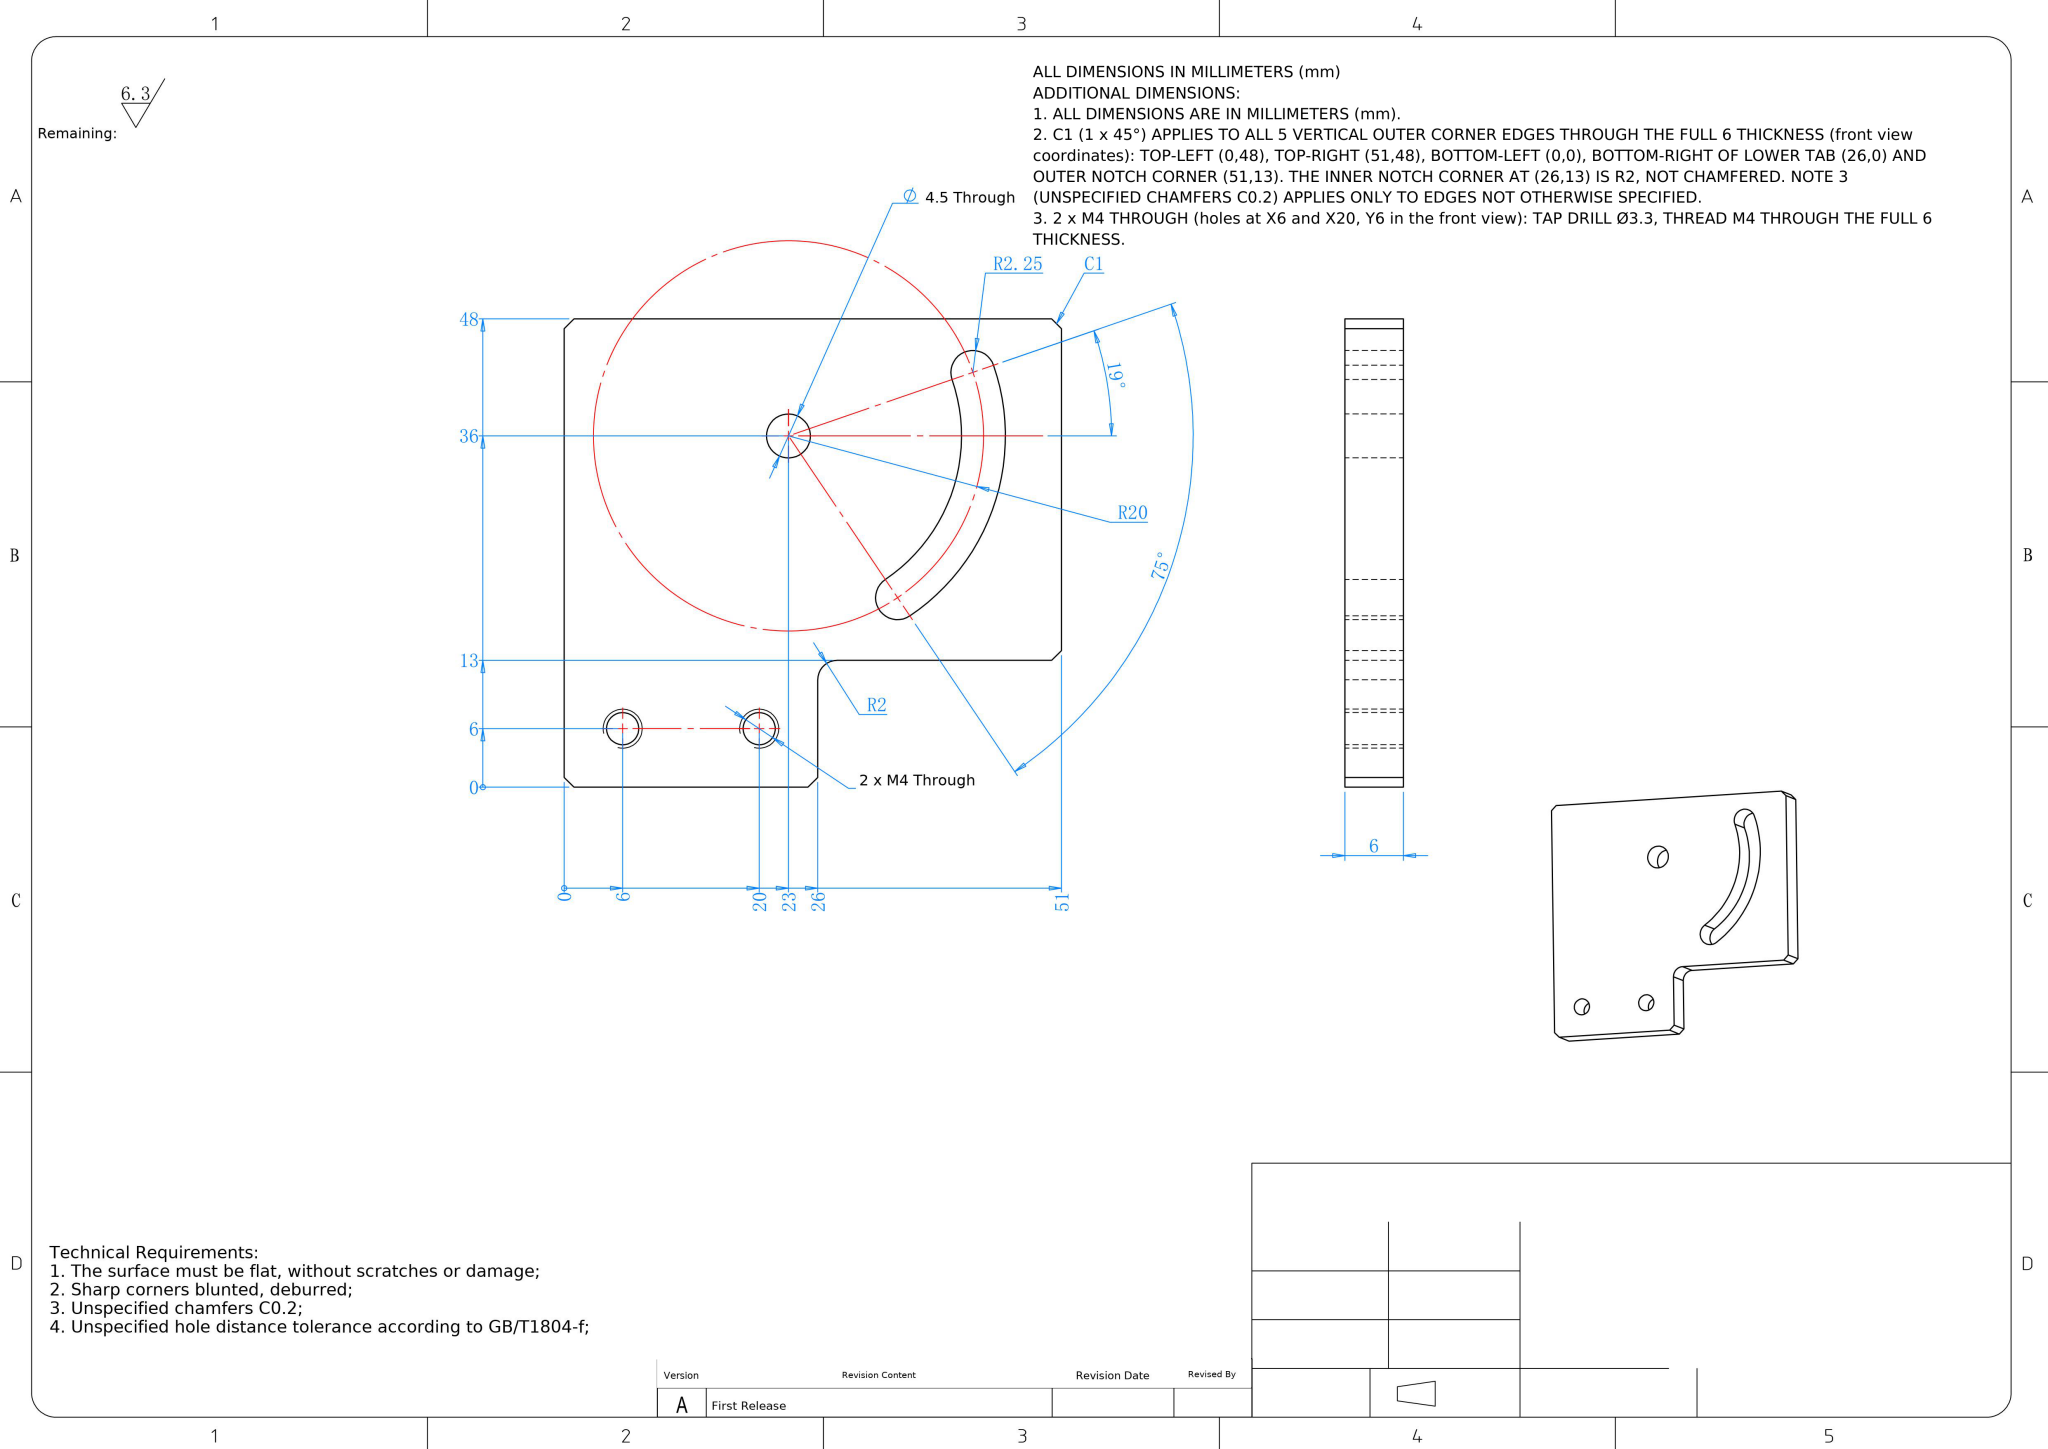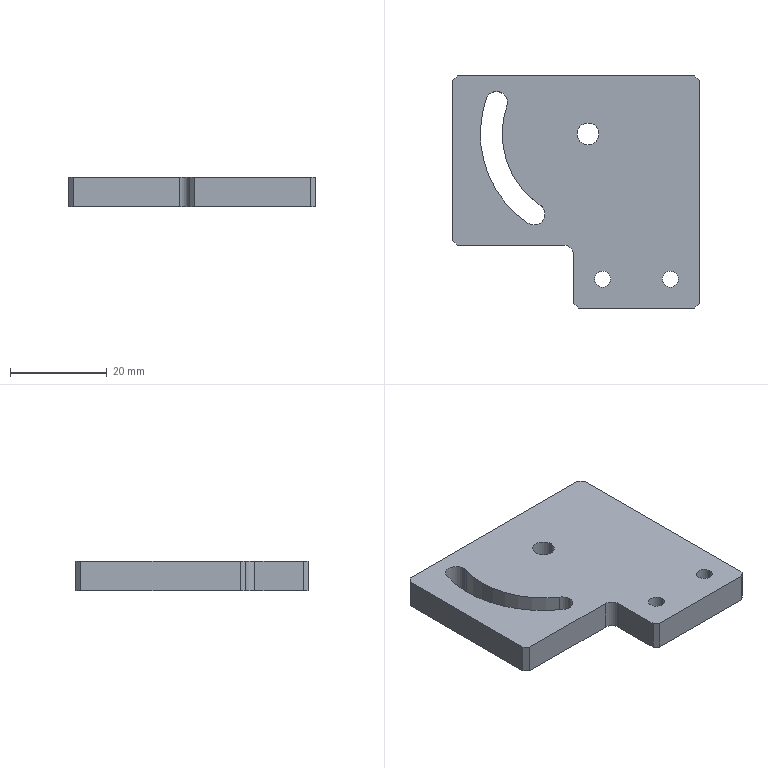Part | NX | mm | Right-Angle Hooked Shelf Bracket 48mm | 1 solid | 26 faces | box 51 x 48 x 6 mm | volume 11728 mm3 | cylinder 13 | plane 13 | commonest cylinder face diameters 4.5 x6 3.3 x4 35.5 x1 44.5 x1 4 x1
STEP:
#1=COLOUR_RGB('',0.7922,0.8196,0.9333);
#2=FILL_AREA_STYLE_COLOUR('',#1);
#3=FILL_AREA_STYLE('',(#2));
#4=SURFACE_STYLE_FILL_AREA(#3);
#5=SURFACE_SIDE_STYLE('',(#4));
#6=SURFACE_STYLE_USAGE(.BOTH.,#5);
#7=PRESENTATION_STYLE_ASSIGNMENT((#6));
#8=CARTESIAN_POINT('',(1.35,-30.,0.));
#9=VERTEX_POINT('',#8);
#10=CARTESIAN_POINT('',(4.65,-30.,0.));
#11=VERTEX_POINT('',#10);
#12=CARTESIAN_POINT('',(3.,-30.,0.));
#13=DIRECTION('',(0.,0.,1.));
#14=DIRECTION('',(1.,0.,0.));
#15=AXIS2_PLACEMENT_3D('',#12,#13,#14);
#16=CIRCLE('',#15,1.65);
#17=EDGE_CURVE('',#9,#11,#16,.T.);
#18=ORIENTED_EDGE('',*,*,#17,.F.);
#19=CARTESIAN_POINT('',(1.35,-30.,6.));
#20=VERTEX_POINT('',#19);
#21=CARTESIAN_POINT('',(1.35,-30.,6.));
#22=DIRECTION('',(0.,0.,1.));
#23=VECTOR('',#22,1000.);
#24=LINE('',#21,#23);
#25=EDGE_CURVE('',#9,#20,#24,.T.);
#26=ORIENTED_EDGE('',*,*,#25,.T.);
#27=CARTESIAN_POINT('',(4.65,-30.,6.));
#28=VERTEX_POINT('',#27);
#29=CARTESIAN_POINT('',(3.,-30.,6.));
#30=DIRECTION('',(0.,0.,1.));
#31=DIRECTION('',(1.,0.,0.));
#32=AXIS2_PLACEMENT_3D('',#29,#30,#31);
#33=CIRCLE('',#32,1.65);
#34=EDGE_CURVE('',#20,#28,#33,.T.);
#35=ORIENTED_EDGE('',*,*,#34,.T.);
#36=CARTESIAN_POINT('',(4.65,-30.,6.));
#37=DIRECTION('',(0.,0.,1.));
#38=VECTOR('',#37,1000.);
#39=LINE('',#36,#38);
#40=EDGE_CURVE('',#11,#28,#39,.T.);
#41=ORIENTED_EDGE('',*,*,#40,.F.);
#42=EDGE_LOOP('',(#18,#26,#35,#41));
#43=FACE_OUTER_BOUND('',#42,.T.);
#44=CARTESIAN_POINT('',(3.,-30.,6.));
#45=DIRECTION('',(0.,0.,1.));
#46=DIRECTION('',(1.,0.,0.));
#47=AXIS2_PLACEMENT_3D('',#44,#45,#46);
#48=CYLINDRICAL_SURFACE('',#47,1.65);
#49=ADVANCED_FACE('',(#43),#48,.F.);
#50=CARTESIAN_POINT('',(15.35,-30.,0.));
#51=VERTEX_POINT('',#50);
#52=CARTESIAN_POINT('',(18.65,-30.,0.));
#53=VERTEX_POINT('',#52);
#54=CARTESIAN_POINT('',(17.,-30.,0.));
#55=DIRECTION('',(0.,0.,1.));
#56=DIRECTION('',(1.,0.,0.));
#57=AXIS2_PLACEMENT_3D('',#54,#55,#56);
#58=CIRCLE('',#57,1.65);
#59=EDGE_CURVE('',#51,#53,#58,.T.);
#60=ORIENTED_EDGE('',*,*,#59,.F.);
#61=CARTESIAN_POINT('',(15.35,-30.,6.));
#62=VERTEX_POINT('',#61);
#63=CARTESIAN_POINT('',(15.35,-30.,6.));
#64=DIRECTION('',(0.,0.,1.));
#65=VECTOR('',#64,1000.);
#66=LINE('',#63,#65);
#67=EDGE_CURVE('',#51,#62,#66,.T.);
#68=ORIENTED_EDGE('',*,*,#67,.T.);
#69=CARTESIAN_POINT('',(18.65,-30.,6.));
#70=VERTEX_POINT('',#69);
#71=CARTESIAN_POINT('',(17.,-30.,6.));
#72=DIRECTION('',(0.,0.,1.));
#73=DIRECTION('',(1.,0.,0.));
#74=AXIS2_PLACEMENT_3D('',#71,#72,#73);
#75=CIRCLE('',#74,1.65);
#76=EDGE_CURVE('',#62,#70,#75,.T.);
#77=ORIENTED_EDGE('',*,*,#76,.T.);
#78=CARTESIAN_POINT('',(18.65,-30.,6.));
#79=DIRECTION('',(0.,0.,1.));
#80=VECTOR('',#79,1000.);
#81=LINE('',#78,#80);
#82=EDGE_CURVE('',#53,#70,#81,.T.);
#83=ORIENTED_EDGE('',*,*,#82,.F.);
#84=EDGE_LOOP('',(#60,#68,#77,#83));
#85=FACE_OUTER_BOUND('',#84,.T.);
#86=CARTESIAN_POINT('',(17.,-30.,6.));
#87=DIRECTION('',(0.,0.,1.));
#88=DIRECTION('',(1.,0.,0.));
#89=AXIS2_PLACEMENT_3D('',#86,#87,#88);
#90=CYLINDRICAL_SURFACE('',#89,1.65);
#91=ADVANCED_FACE('',(#85),#90,.F.);
#92=CARTESIAN_POINT('',(-8.934,-16.581,0.));
#93=VERTEX_POINT('',#92);
#94=CARTESIAN_POINT('',(-9.926,-14.715,0.));
#95=VERTEX_POINT('',#94);
#96=CARTESIAN_POINT('',(-11.184,-16.581,0.));
#97=DIRECTION('',(0.,0.,1.));
#98=DIRECTION('',(-1.,0.,0.));
#99=AXIS2_PLACEMENT_3D('',#96,#97,#98);
#100=CIRCLE('',#99,2.25);
#101=EDGE_CURVE('',#93,#95,#100,.T.);
#102=ORIENTED_EDGE('',*,*,#101,.F.);
#103=CARTESIAN_POINT('',(-8.934,-16.581,6.));
#104=VERTEX_POINT('',#103);
#105=CARTESIAN_POINT('',(-8.934,-16.581,0.));
#106=DIRECTION('',(0.,0.,1.));
#107=VECTOR('',#106,1000.);
#108=LINE('',#105,#107);
#109=EDGE_CURVE('',#93,#104,#108,.T.);
#110=ORIENTED_EDGE('',*,*,#109,.T.);
#111=CARTESIAN_POINT('',(-9.926,-14.715,6.));
#112=VERTEX_POINT('',#111);
#113=CARTESIAN_POINT('',(-11.184,-16.581,6.));
#114=DIRECTION('',(0.,0.,1.));
#115=DIRECTION('',(-1.,0.,0.));
#116=AXIS2_PLACEMENT_3D('',#113,#114,#115);
#117=CIRCLE('',#116,2.25);
#118=EDGE_CURVE('',#104,#112,#117,.T.);
#119=ORIENTED_EDGE('',*,*,#118,.T.);
#120=CARTESIAN_POINT('',(-9.926,-14.715,0.));
#121=DIRECTION('',(0.,0.,1.));
#122=VECTOR('',#121,1000.);
#123=LINE('',#120,#122);
#124=EDGE_CURVE('',#95,#112,#123,.T.);
#125=ORIENTED_EDGE('',*,*,#124,.F.);
#126=EDGE_LOOP('',(#102,#110,#119,#125));
#127=FACE_OUTER_BOUND('',#126,.T.);
#128=CARTESIAN_POINT('',(-11.184,-16.581,0.));
#129=DIRECTION('',(0.,0.,1.));
#130=DIRECTION('',(1.,0.,0.));
#131=AXIS2_PLACEMENT_3D('',#128,#129,#130);
#132=CYLINDRICAL_SURFACE('',#131,2.25);
#133=ADVANCED_FACE('',(#127),#132,.F.);
#134=CARTESIAN_POINT('',(-16.66,6.511,0.));
#135=VERTEX_POINT('',#134);
#136=CARTESIAN_POINT('',(-21.038,7.244,0.));
#137=VERTEX_POINT('',#136);
#138=CARTESIAN_POINT('',(-18.91,6.511,0.));
#139=DIRECTION('',(0.,0.,1.));
#140=DIRECTION('',(1.,0.,0.));
#141=AXIS2_PLACEMENT_3D('',#138,#139,#140);
#142=CIRCLE('',#141,2.25);
#143=EDGE_CURVE('',#135,#137,#142,.T.);
#144=ORIENTED_EDGE('',*,*,#143,.F.);
#145=CARTESIAN_POINT('',(-16.66,6.511,6.));
#146=VERTEX_POINT('',#145);
#147=CARTESIAN_POINT('',(-16.66,6.511,0.));
#148=DIRECTION('',(0.,0.,1.));
#149=VECTOR('',#148,1000.);
#150=LINE('',#147,#149);
#151=EDGE_CURVE('',#135,#146,#150,.T.);
#152=ORIENTED_EDGE('',*,*,#151,.T.);
#153=CARTESIAN_POINT('',(-21.038,7.244,6.));
#154=VERTEX_POINT('',#153);
#155=CARTESIAN_POINT('',(-18.91,6.511,6.));
#156=DIRECTION('',(0.,0.,1.));
#157=DIRECTION('',(1.,0.,0.));
#158=AXIS2_PLACEMENT_3D('',#155,#156,#157);
#159=CIRCLE('',#158,2.25);
#160=EDGE_CURVE('',#146,#154,#159,.T.);
#161=ORIENTED_EDGE('',*,*,#160,.T.);
#162=CARTESIAN_POINT('',(-21.038,7.244,0.));
#163=DIRECTION('',(0.,0.,1.));
#164=VECTOR('',#163,1000.);
#165=LINE('',#162,#164);
#166=EDGE_CURVE('',#137,#154,#165,.T.);
#167=ORIENTED_EDGE('',*,*,#166,.F.);
#168=EDGE_LOOP('',(#144,#152,#161,#167));
#169=FACE_OUTER_BOUND('',#168,.T.);
#170=CARTESIAN_POINT('',(-18.91,6.511,0.));
#171=DIRECTION('',(0.,0.,1.));
#172=DIRECTION('',(1.,0.,0.));
#173=AXIS2_PLACEMENT_3D('',#170,#171,#172);
#174=CYLINDRICAL_SURFACE('',#173,2.25);
#175=ADVANCED_FACE('',(#169),#174,.F.);
#176=CARTESIAN_POINT('',(-2.25,0.,0.));
#177=VERTEX_POINT('',#176);
#178=CARTESIAN_POINT('',(2.25,0.,0.));
#179=VERTEX_POINT('',#178);
#180=CARTESIAN_POINT('',(0.,0.,0.));
#181=DIRECTION('',(0.,0.,1.));
#182=DIRECTION('',(1.,0.,0.));
#183=AXIS2_PLACEMENT_3D('',#180,#181,#182);
#184=CIRCLE('',#183,2.25);
#185=EDGE_CURVE('',#177,#179,#184,.T.);
#186=ORIENTED_EDGE('',*,*,#185,.F.);
#187=CARTESIAN_POINT('',(-2.25,0.,6.));
#188=VERTEX_POINT('',#187);
#189=CARTESIAN_POINT('',(-2.25,0.,6.));
#190=DIRECTION('',(0.,0.,1.));
#191=VECTOR('',#190,1000.);
#192=LINE('',#189,#191);
#193=EDGE_CURVE('',#177,#188,#192,.T.);
#194=ORIENTED_EDGE('',*,*,#193,.T.);
#195=CARTESIAN_POINT('',(2.25,0.,6.));
#196=VERTEX_POINT('',#195);
#197=CARTESIAN_POINT('',(0.,0.,6.));
#198=DIRECTION('',(0.,0.,1.));
#199=DIRECTION('',(1.,0.,0.));
#200=AXIS2_PLACEMENT_3D('',#197,#198,#199);
#201=CIRCLE('',#200,2.25);
#202=EDGE_CURVE('',#188,#196,#201,.T.);
#203=ORIENTED_EDGE('',*,*,#202,.T.);
#204=CARTESIAN_POINT('',(2.25,0.,6.));
#205=DIRECTION('',(0.,0.,1.));
#206=VECTOR('',#205,1000.);
#207=LINE('',#204,#206);
#208=EDGE_CURVE('',#179,#196,#207,.T.);
#209=ORIENTED_EDGE('',*,*,#208,.F.);
#210=EDGE_LOOP('',(#186,#194,#203,#209));
#211=FACE_OUTER_BOUND('',#210,.T.);
#212=CARTESIAN_POINT('',(0.,0.,6.));
#213=DIRECTION('',(0.,0.,1.));
#214=DIRECTION('',(1.,0.,0.));
#215=AXIS2_PLACEMENT_3D('',#212,#213,#214);
#216=CYLINDRICAL_SURFACE('',#215,2.25);
#217=ADVANCED_FACE('',(#211),#216,.F.);
#218=CARTESIAN_POINT('',(-28.,11.,6.));
#219=VERTEX_POINT('',#218);
#220=CARTESIAN_POINT('',(-28.,-22.,6.));
#221=VERTEX_POINT('',#220);
#222=CARTESIAN_POINT('',(-28.,12.,6.));
#223=DIRECTION('',(0.,-1.,0.));
#224=VECTOR('',#223,1000.);
#225=LINE('',#222,#224);
#226=EDGE_CURVE('',#219,#221,#225,.T.);
#227=ORIENTED_EDGE('',*,*,#226,.F.);
#228=CARTESIAN_POINT('',(-28.,11.,0.));
#229=VERTEX_POINT('',#228);
#230=CARTESIAN_POINT('',(-28.,11.,6.));
#231=DIRECTION('',(0.,0.,-1.));
#232=VECTOR('',#231,1000.);
#233=LINE('',#230,#232);
#234=EDGE_CURVE('',#219,#229,#233,.T.);
#235=ORIENTED_EDGE('',*,*,#234,.T.);
#236=CARTESIAN_POINT('',(-28.,-22.,0.));
#237=VERTEX_POINT('',#236);
#238=CARTESIAN_POINT('',(-28.,12.,0.));
#239=DIRECTION('',(0.,-1.,0.));
#240=VECTOR('',#239,1000.);
#241=LINE('',#238,#240);
#242=EDGE_CURVE('',#229,#237,#241,.T.);
#243=ORIENTED_EDGE('',*,*,#242,.T.);
#244=CARTESIAN_POINT('',(-28.,-22.,6.));
#245=DIRECTION('',(0.,0.,1.));
#246=VECTOR('',#245,1000.);
#247=LINE('',#244,#246);
#248=EDGE_CURVE('',#237,#221,#247,.T.);
#249=ORIENTED_EDGE('',*,*,#248,.T.);
#250=EDGE_LOOP('',(#227,#235,#243,#249));
#251=FACE_OUTER_BOUND('',#250,.T.);
#252=CARTESIAN_POINT('',(-28.,12.,6.));
#253=DIRECTION('',(1.,0.,0.));
#254=DIRECTION('',(-0.,1.,0.));
#255=AXIS2_PLACEMENT_3D('',#252,#253,#254);
#256=PLANE('',#255);
#257=ADVANCED_FACE('',(#251),#256,.F.);
#258=CARTESIAN_POINT('',(-2.,-36.,0.));
#259=VERTEX_POINT('',#258);
#260=CARTESIAN_POINT('',(22.,-36.,0.));
#261=VERTEX_POINT('',#260);
#262=CARTESIAN_POINT('',(-28.,-36.,0.));
#263=DIRECTION('',(1.,0.,0.));
#264=VECTOR('',#263,1000.);
#265=LINE('',#262,#264);
#266=EDGE_CURVE('',#259,#261,#265,.T.);
#267=ORIENTED_EDGE('',*,*,#266,.T.);
#268=CARTESIAN_POINT('',(22.,-36.,6.));
#269=VERTEX_POINT('',#268);
#270=CARTESIAN_POINT('',(22.,-36.,6.));
#271=DIRECTION('',(0.,0.,1.));
#272=VECTOR('',#271,1000.);
#273=LINE('',#270,#272);
#274=EDGE_CURVE('',#261,#269,#273,.T.);
#275=ORIENTED_EDGE('',*,*,#274,.T.);
#276=CARTESIAN_POINT('',(-2.,-36.,6.));
#277=VERTEX_POINT('',#276);
#278=CARTESIAN_POINT('',(-28.,-36.,6.));
#279=DIRECTION('',(1.,0.,0.));
#280=VECTOR('',#279,1000.);
#281=LINE('',#278,#280);
#282=EDGE_CURVE('',#277,#269,#281,.T.);
#283=ORIENTED_EDGE('',*,*,#282,.F.);
#284=CARTESIAN_POINT('',(-2.,-36.,6.));
#285=DIRECTION('',(0.,0.,-1.));
#286=VECTOR('',#285,1000.);
#287=LINE('',#284,#286);
#288=EDGE_CURVE('',#277,#259,#287,.T.);
#289=ORIENTED_EDGE('',*,*,#288,.T.);
#290=EDGE_LOOP('',(#267,#275,#283,#289));
#291=FACE_OUTER_BOUND('',#290,.T.);
#292=CARTESIAN_POINT('',(-28.,-36.,6.));
#293=DIRECTION('',(0.,1.,0.));
#294=DIRECTION('',(0.,0.,1.));
#295=AXIS2_PLACEMENT_3D('',#292,#293,#294);
#296=PLANE('',#295);
#297=ADVANCED_FACE('',(#291),#296,.F.);
#298=CARTESIAN_POINT('',(23.,-35.,0.));
#299=VERTEX_POINT('',#298);
#300=CARTESIAN_POINT('',(23.,11.,0.));
#301=VERTEX_POINT('',#300);
#302=CARTESIAN_POINT('',(23.,12.,0.));
#303=DIRECTION('',(0.,1.,0.));
#304=VECTOR('',#303,1000.);
#305=LINE('',#302,#304);
#306=EDGE_CURVE('',#299,#301,#305,.T.);
#307=ORIENTED_EDGE('',*,*,#306,.T.);
#308=CARTESIAN_POINT('',(23.,11.,6.));
#309=VERTEX_POINT('',#308);
#310=CARTESIAN_POINT('',(23.,11.,6.));
#311=DIRECTION('',(0.,0.,1.));
#312=VECTOR('',#311,1000.);
#313=LINE('',#310,#312);
#314=EDGE_CURVE('',#301,#309,#313,.T.);
#315=ORIENTED_EDGE('',*,*,#314,.T.);
#316=CARTESIAN_POINT('',(23.,-35.,6.));
#317=VERTEX_POINT('',#316);
#318=CARTESIAN_POINT('',(23.,12.,6.));
#319=DIRECTION('',(0.,1.,0.));
#320=VECTOR('',#319,1000.);
#321=LINE('',#318,#320);
#322=EDGE_CURVE('',#317,#309,#321,.T.);
#323=ORIENTED_EDGE('',*,*,#322,.F.);
#324=CARTESIAN_POINT('',(23.,-35.,6.));
#325=DIRECTION('',(0.,0.,-1.));
#326=VECTOR('',#325,1000.);
#327=LINE('',#324,#326);
#328=EDGE_CURVE('',#317,#299,#327,.T.);
#329=ORIENTED_EDGE('',*,*,#328,.T.);
#330=EDGE_LOOP('',(#307,#315,#323,#329));
#331=FACE_OUTER_BOUND('',#330,.T.);
#332=CARTESIAN_POINT('',(23.,12.,6.));
#333=DIRECTION('',(-1.,0.,0.));
#334=DIRECTION('',(0.,0.,1.));
#335=AXIS2_PLACEMENT_3D('',#332,#333,#334);
#336=PLANE('',#335);
#337=ADVANCED_FACE('',(#331),#336,.F.);
#338=CARTESIAN_POINT('',(22.,12.,0.));
#339=VERTEX_POINT('',#338);
#340=CARTESIAN_POINT('',(-27.,12.,0.));
#341=VERTEX_POINT('',#340);
#342=CARTESIAN_POINT('',(-28.,12.,0.));
#343=DIRECTION('',(-1.,0.,0.));
#344=VECTOR('',#343,1000.);
#345=LINE('',#342,#344);
#346=EDGE_CURVE('',#339,#341,#345,.T.);
#347=ORIENTED_EDGE('',*,*,#346,.T.);
#348=CARTESIAN_POINT('',(-27.,12.,6.));
#349=VERTEX_POINT('',#348);
#350=CARTESIAN_POINT('',(-27.,12.,6.));
#351=DIRECTION('',(0.,0.,1.));
#352=VECTOR('',#351,1000.);
#353=LINE('',#350,#352);
#354=EDGE_CURVE('',#341,#349,#353,.T.);
#355=ORIENTED_EDGE('',*,*,#354,.T.);
#356=CARTESIAN_POINT('',(22.,12.,6.));
#357=VERTEX_POINT('',#356);
#358=CARTESIAN_POINT('',(-28.,12.,6.));
#359=DIRECTION('',(-1.,0.,0.));
#360=VECTOR('',#359,1000.);
#361=LINE('',#358,#360);
#362=EDGE_CURVE('',#357,#349,#361,.T.);
#363=ORIENTED_EDGE('',*,*,#362,.F.);
#364=CARTESIAN_POINT('',(22.,12.,6.));
#365=DIRECTION('',(0.,0.,-1.));
#366=VECTOR('',#365,1000.);
#367=LINE('',#364,#366);
#368=EDGE_CURVE('',#357,#339,#367,.T.);
#369=ORIENTED_EDGE('',*,*,#368,.T.);
#370=EDGE_LOOP('',(#347,#355,#363,#369));
#371=FACE_OUTER_BOUND('',#370,.T.);
#372=CARTESIAN_POINT('',(-28.,12.,6.));
#373=DIRECTION('',(0.,-1.,0.));
#374=DIRECTION('',(0.,0.,-1.));
#375=AXIS2_PLACEMENT_3D('',#372,#373,#374);
#376=PLANE('',#375);
#377=ADVANCED_FACE('',(#371),#376,.F.);
#378=ORIENTED_EDGE('',*,*,#362,.T.);
#379=CARTESIAN_POINT('',(-19.5,19.5,6.));
#380=DIRECTION('',(-0.7071,-0.7071,0.));
#381=VECTOR('',#380,1000.);
#382=LINE('',#379,#381);
#383=EDGE_CURVE('',#349,#219,#382,.T.);
#384=ORIENTED_EDGE('',*,*,#383,.T.);
#385=ORIENTED_EDGE('',*,*,#226,.T.);
#386=CARTESIAN_POINT('',(-27.,-23.,6.));
#387=VERTEX_POINT('',#386);
#388=CARTESIAN_POINT('',(-25.,-25.,6.));
#389=DIRECTION('',(0.7071,-0.7071,0.));
#390=VECTOR('',#389,1000.);
#391=LINE('',#388,#390);
#392=EDGE_CURVE('',#221,#387,#391,.T.);
#393=ORIENTED_EDGE('',*,*,#392,.T.);
#394=CARTESIAN_POINT('',(-5.,-23.,6.));
#395=VERTEX_POINT('',#394);
#396=CARTESIAN_POINT('',(-28.,-23.,6.));
#397=DIRECTION('',(-1.,0.,0.));
#398=VECTOR('',#397,1000.);
#399=LINE('',#396,#398);
#400=EDGE_CURVE('',#395,#387,#399,.T.);
#401=ORIENTED_EDGE('',*,*,#400,.F.);
#402=CARTESIAN_POINT('',(-3.,-25.,6.));
#403=VERTEX_POINT('',#402);
#404=CARTESIAN_POINT('',(-5.,-25.,6.));
#405=DIRECTION('',(0.,0.,1.));
#406=DIRECTION('',(-1.,0.,0.));
#407=AXIS2_PLACEMENT_3D('',#404,#405,#406);
#408=CIRCLE('',#407,2.);
#409=EDGE_CURVE('',#403,#395,#408,.T.);
#410=ORIENTED_EDGE('',*,*,#409,.F.);
#411=CARTESIAN_POINT('',(-3.,-35.,6.));
#412=VERTEX_POINT('',#411);
#413=CARTESIAN_POINT('',(-3.,-36.,6.));
#414=DIRECTION('',(0.,1.,0.));
#415=VECTOR('',#414,1000.);
#416=LINE('',#413,#415);
#417=EDGE_CURVE('',#412,#403,#416,.T.);
#418=ORIENTED_EDGE('',*,*,#417,.F.);
#419=CARTESIAN_POINT('',(-19.,-19.,6.));
#420=DIRECTION('',(0.7071,-0.7071,0.));
#421=VECTOR('',#420,1000.);
#422=LINE('',#419,#421);
#423=EDGE_CURVE('',#412,#277,#422,.T.);
#424=ORIENTED_EDGE('',*,*,#423,.T.);
#425=ORIENTED_EDGE('',*,*,#282,.T.);
#426=CARTESIAN_POINT('',(29.,-29.,6.));
#427=DIRECTION('',(0.7071,0.7071,0.));
#428=VECTOR('',#427,1000.);
#429=LINE('',#426,#428);
#430=EDGE_CURVE('',#269,#317,#429,.T.);
#431=ORIENTED_EDGE('',*,*,#430,.T.);
#432=ORIENTED_EDGE('',*,*,#322,.T.);
#433=CARTESIAN_POINT('',(17.,17.,6.));
#434=DIRECTION('',(-0.7071,0.7071,0.));
#435=VECTOR('',#434,1000.);
#436=LINE('',#433,#435);
#437=EDGE_CURVE('',#309,#357,#436,.T.);
#438=ORIENTED_EDGE('',*,*,#437,.T.);
#439=EDGE_LOOP('',(#378,#384,#385,#393,#401,#410,#418,#424,#425,#431,#432,#438));
#440=FACE_OUTER_BOUND('',#439,.T.);
#441=CARTESIAN_POINT('',(3.,-30.,6.));
#442=DIRECTION('',(0.,0.,1.));
#443=DIRECTION('',(1.,0.,0.));
#444=AXIS2_PLACEMENT_3D('',#441,#442,#443);
#445=CIRCLE('',#444,1.65);
#446=EDGE_CURVE('',#28,#20,#445,.T.);
#447=ORIENTED_EDGE('',*,*,#446,.F.);
#448=ORIENTED_EDGE('',*,*,#34,.F.);
#449=EDGE_LOOP('',(#447,#448));
#450=FACE_BOUND('',#449,.T.);
#451=CARTESIAN_POINT('',(17.,-30.,6.));
#452=DIRECTION('',(0.,0.,1.));
#453=DIRECTION('',(1.,0.,0.));
#454=AXIS2_PLACEMENT_3D('',#451,#452,#453);
#455=CIRCLE('',#454,1.65);
#456=EDGE_CURVE('',#70,#62,#455,.T.);
#457=ORIENTED_EDGE('',*,*,#456,.F.);
#458=ORIENTED_EDGE('',*,*,#76,.F.);
#459=EDGE_LOOP('',(#457,#458));
#460=FACE_BOUND('',#459,.T.);
#461=CARTESIAN_POINT('',(-16.783,5.779,6.));
#462=VERTEX_POINT('',#461);
#463=CARTESIAN_POINT('',(-18.91,6.511,6.));
#464=DIRECTION('',(0.,0.,1.));
#465=DIRECTION('',(1.,0.,0.));
#466=AXIS2_PLACEMENT_3D('',#463,#464,#465);
#467=CIRCLE('',#466,2.25);
#468=EDGE_CURVE('',#462,#146,#467,.T.);
#469=ORIENTED_EDGE('',*,*,#468,.F.);
#470=CARTESIAN_POINT('',(0.,0.,6.));
#471=DIRECTION('',(0.,0.,-1.));
#472=DIRECTION('',(1.,0.,0.));
#473=AXIS2_PLACEMENT_3D('',#470,#471,#472);
#474=CIRCLE('',#473,17.75);
#475=EDGE_CURVE('',#112,#462,#474,.T.);
#476=ORIENTED_EDGE('',*,*,#475,.F.);
#477=ORIENTED_EDGE('',*,*,#118,.F.);
#478=CARTESIAN_POINT('',(-12.442,-18.446,6.));
#479=VERTEX_POINT('',#478);
#480=CARTESIAN_POINT('',(-11.184,-16.581,6.));
#481=DIRECTION('',(0.,0.,1.));
#482=DIRECTION('',(-1.,0.,0.));
#483=AXIS2_PLACEMENT_3D('',#480,#481,#482);
#484=CIRCLE('',#483,2.25);
#485=EDGE_CURVE('',#479,#104,#484,.T.);
#486=ORIENTED_EDGE('',*,*,#485,.F.);
#487=CARTESIAN_POINT('',(0.,0.,6.));
#488=DIRECTION('',(0.,0.,1.));
#489=DIRECTION('',(1.,0.,0.));
#490=AXIS2_PLACEMENT_3D('',#487,#488,#489);
#491=CIRCLE('',#490,22.25);
#492=EDGE_CURVE('',#154,#479,#491,.T.);
#493=ORIENTED_EDGE('',*,*,#492,.F.);
#494=ORIENTED_EDGE('',*,*,#160,.F.);
#495=EDGE_LOOP('',(#469,#476,#477,#486,#493,#494));
#496=FACE_BOUND('',#495,.T.);
#497=CARTESIAN_POINT('',(0.,0.,6.));
#498=DIRECTION('',(0.,0.,1.));
#499=DIRECTION('',(1.,0.,0.));
#500=AXIS2_PLACEMENT_3D('',#497,#498,#499);
#501=CIRCLE('',#500,2.25);
#502=EDGE_CURVE('',#196,#188,#501,.T.);
#503=ORIENTED_EDGE('',*,*,#502,.F.);
#504=ORIENTED_EDGE('',*,*,#202,.F.);
#505=EDGE_LOOP('',(#503,#504));
#506=FACE_BOUND('',#505,.T.);
#507=CARTESIAN_POINT('',(0.,0.,6.));
#508=DIRECTION('',(0.,0.,1.));
#509=DIRECTION('',(1.,0.,0.));
#510=AXIS2_PLACEMENT_3D('',#507,#508,#509);
#511=PLANE('',#510);
#512=ADVANCED_FACE('',(#440,#450,#460,#496,#506),#511,.T.);
#513=CARTESIAN_POINT('',(3.,-30.,0.));
#514=DIRECTION('',(0.,0.,1.));
#515=DIRECTION('',(1.,0.,0.));
#516=AXIS2_PLACEMENT_3D('',#513,#514,#515);
#517=CIRCLE('',#516,1.65);
#518=EDGE_CURVE('',#11,#9,#517,.T.);
#519=ORIENTED_EDGE('',*,*,#518,.T.);
#520=ORIENTED_EDGE('',*,*,#17,.T.);
#521=EDGE_LOOP('',(#519,#520));
#522=FACE_BOUND('',#521,.T.);
#523=CARTESIAN_POINT('',(17.,-30.,0.));
#524=DIRECTION('',(0.,0.,1.));
#525=DIRECTION('',(1.,0.,0.));
#526=AXIS2_PLACEMENT_3D('',#523,#524,#525);
#527=CIRCLE('',#526,1.65);
#528=EDGE_CURVE('',#53,#51,#527,.T.);
#529=ORIENTED_EDGE('',*,*,#528,.T.);
#530=ORIENTED_EDGE('',*,*,#59,.T.);
#531=EDGE_LOOP('',(#529,#530));
#532=FACE_BOUND('',#531,.T.);
#533=CARTESIAN_POINT('',(-16.783,5.779,0.));
#534=VERTEX_POINT('',#533);
#535=CARTESIAN_POINT('',(0.,0.,0.));
#536=DIRECTION('',(0.,0.,-1.));
#537=DIRECTION('',(1.,0.,0.));
#538=AXIS2_PLACEMENT_3D('',#535,#536,#537);
#539=CIRCLE('',#538,17.75);
#540=EDGE_CURVE('',#95,#534,#539,.T.);
#541=ORIENTED_EDGE('',*,*,#540,.T.);
#542=CARTESIAN_POINT('',(-18.91,6.511,0.));
#543=DIRECTION('',(0.,0.,1.));
#544=DIRECTION('',(1.,0.,0.));
#545=AXIS2_PLACEMENT_3D('',#542,#543,#544);
#546=CIRCLE('',#545,2.25);
#547=EDGE_CURVE('',#534,#135,#546,.T.);
#548=ORIENTED_EDGE('',*,*,#547,.T.);
#549=ORIENTED_EDGE('',*,*,#143,.T.);
#550=CARTESIAN_POINT('',(-12.442,-18.446,0.));
#551=VERTEX_POINT('',#550);
#552=CARTESIAN_POINT('',(0.,0.,0.));
#553=DIRECTION('',(0.,0.,1.));
#554=DIRECTION('',(1.,0.,0.));
#555=AXIS2_PLACEMENT_3D('',#552,#553,#554);
#556=CIRCLE('',#555,22.25);
#557=EDGE_CURVE('',#137,#551,#556,.T.);
#558=ORIENTED_EDGE('',*,*,#557,.T.);
#559=CARTESIAN_POINT('',(-11.184,-16.581,0.));
#560=DIRECTION('',(0.,0.,1.));
#561=DIRECTION('',(-1.,0.,0.));
#562=AXIS2_PLACEMENT_3D('',#559,#560,#561);
#563=CIRCLE('',#562,2.25);
#564=EDGE_CURVE('',#551,#93,#563,.T.);
#565=ORIENTED_EDGE('',*,*,#564,.T.);
#566=ORIENTED_EDGE('',*,*,#101,.T.);
#567=EDGE_LOOP('',(#541,#548,#549,#558,#565,#566));
#568=FACE_BOUND('',#567,.T.);
#569=CARTESIAN_POINT('',(0.,0.,0.));
#570=DIRECTION('',(0.,0.,1.));
#571=DIRECTION('',(1.,0.,0.));
#572=AXIS2_PLACEMENT_3D('',#569,#570,#571);
#573=CIRCLE('',#572,2.25);
#574=EDGE_CURVE('',#179,#177,#573,.T.);
#575=ORIENTED_EDGE('',*,*,#574,.T.);
#576=ORIENTED_EDGE('',*,*,#185,.T.);
#577=EDGE_LOOP('',(#575,#576));
#578=FACE_BOUND('',#577,.T.);
#579=ORIENTED_EDGE('',*,*,#242,.F.);
#580=CARTESIAN_POINT('',(-28.,11.,0.));
#581=DIRECTION('',(0.7071,0.7071,0.));
#582=VECTOR('',#581,1000.);
#583=LINE('',#580,#582);
#584=EDGE_CURVE('',#229,#341,#583,.T.);
#585=ORIENTED_EDGE('',*,*,#584,.T.);
#586=ORIENTED_EDGE('',*,*,#346,.F.);
#587=CARTESIAN_POINT('',(22.,12.,0.));
#588=DIRECTION('',(0.7071,-0.7071,0.));
#589=VECTOR('',#588,1000.);
#590=LINE('',#587,#589);
#591=EDGE_CURVE('',#339,#301,#590,.T.);
#592=ORIENTED_EDGE('',*,*,#591,.T.);
#593=ORIENTED_EDGE('',*,*,#306,.F.);
#594=CARTESIAN_POINT('',(23.,-35.,0.));
#595=DIRECTION('',(-0.7071,-0.7071,0.));
#596=VECTOR('',#595,1000.);
#597=LINE('',#594,#596);
#598=EDGE_CURVE('',#299,#261,#597,.T.);
#599=ORIENTED_EDGE('',*,*,#598,.T.);
#600=ORIENTED_EDGE('',*,*,#266,.F.);
#601=CARTESIAN_POINT('',(-3.,-35.,0.));
#602=VERTEX_POINT('',#601);
#603=CARTESIAN_POINT('',(-3.,-35.,0.));
#604=DIRECTION('',(-0.7071,0.7071,0.));
#605=VECTOR('',#604,1000.);
#606=LINE('',#603,#605);
#607=EDGE_CURVE('',#259,#602,#606,.T.);
#608=ORIENTED_EDGE('',*,*,#607,.T.);
#609=CARTESIAN_POINT('',(-3.,-25.,0.));
#610=VERTEX_POINT('',#609);
#611=CARTESIAN_POINT('',(-3.,-36.,0.));
#612=DIRECTION('',(0.,1.,0.));
#613=VECTOR('',#612,1000.);
#614=LINE('',#611,#613);
#615=EDGE_CURVE('',#602,#610,#614,.T.);
#616=ORIENTED_EDGE('',*,*,#615,.T.);
#617=CARTESIAN_POINT('',(-5.,-23.,0.));
#618=VERTEX_POINT('',#617);
#619=CARTESIAN_POINT('',(-5.,-25.,0.));
#620=DIRECTION('',(0.,0.,1.));
#621=DIRECTION('',(-1.,0.,0.));
#622=AXIS2_PLACEMENT_3D('',#619,#620,#621);
#623=CIRCLE('',#622,2.);
#624=EDGE_CURVE('',#610,#618,#623,.T.);
#625=ORIENTED_EDGE('',*,*,#624,.T.);
#626=CARTESIAN_POINT('',(-27.,-23.,0.));
#627=VERTEX_POINT('',#626);
#628=CARTESIAN_POINT('',(-28.,-23.,0.));
#629=DIRECTION('',(-1.,0.,0.));
#630=VECTOR('',#629,1000.);
#631=LINE('',#628,#630);
#632=EDGE_CURVE('',#618,#627,#631,.T.);
#633=ORIENTED_EDGE('',*,*,#632,.T.);
#634=CARTESIAN_POINT('',(-28.,-22.,0.));
#635=DIRECTION('',(-0.7071,0.7071,0.));
#636=VECTOR('',#635,1000.);
#637=LINE('',#634,#636);
#638=EDGE_CURVE('',#627,#237,#637,.T.);
#639=ORIENTED_EDGE('',*,*,#638,.T.);
#640=EDGE_LOOP('',(#579,#585,#586,#592,#593,#599,#600,#608,#616,#625,#633,#639));
#641=FACE_OUTER_BOUND('',#640,.T.);
#642=CARTESIAN_POINT('',(0.,0.,0.));
#643=DIRECTION('',(0.,0.,1.));
#644=DIRECTION('',(1.,0.,0.));
#645=AXIS2_PLACEMENT_3D('',#642,#643,#644);
#646=PLANE('',#645);
#647=ADVANCED_FACE('',(#522,#532,#568,#578,#641),#646,.F.);
#648=ORIENTED_EDGE('',*,*,#193,.F.);
#649=ORIENTED_EDGE('',*,*,#574,.F.);
#650=ORIENTED_EDGE('',*,*,#208,.T.);
#651=ORIENTED_EDGE('',*,*,#502,.T.);
#652=EDGE_LOOP('',(#648,#649,#650,#651));
#653=FACE_OUTER_BOUND('',#652,.T.);
#654=CARTESIAN_POINT('',(0.,0.,6.));
#655=DIRECTION('',(0.,0.,1.));
#656=DIRECTION('',(1.,0.,0.));
#657=AXIS2_PLACEMENT_3D('',#654,#655,#656);
#658=CYLINDRICAL_SURFACE('',#657,2.25);
#659=ADVANCED_FACE('',(#653),#658,.F.);
#660=ORIENTED_EDGE('',*,*,#151,.F.);
#661=ORIENTED_EDGE('',*,*,#547,.F.);
#662=CARTESIAN_POINT('',(-16.783,5.779,0.));
#663=DIRECTION('',(0.,0.,1.));
#664=VECTOR('',#663,1000.);
#665=LINE('',#662,#664);
#666=EDGE_CURVE('',#534,#462,#665,.T.);
#667=ORIENTED_EDGE('',*,*,#666,.T.);
#668=ORIENTED_EDGE('',*,*,#468,.T.);
#669=EDGE_LOOP('',(#660,#661,#667,#668));
#670=FACE_OUTER_BOUND('',#669,.T.);
#671=CARTESIAN_POINT('',(-18.91,6.511,0.));
#672=DIRECTION('',(0.,0.,1.));
#673=DIRECTION('',(1.,0.,0.));
#674=AXIS2_PLACEMENT_3D('',#671,#672,#673);
#675=CYLINDRICAL_SURFACE('',#674,2.25);
#676=ADVANCED_FACE('',(#670),#675,.F.);
#677=ORIENTED_EDGE('',*,*,#475,.T.);
#678=ORIENTED_EDGE('',*,*,#666,.F.);
#679=ORIENTED_EDGE('',*,*,#540,.F.);
#680=ORIENTED_EDGE('',*,*,#124,.T.);
#681=EDGE_LOOP('',(#677,#678,#679,#680));
#682=FACE_OUTER_BOUND('',#681,.T.);
#683=CARTESIAN_POINT('',(0.,0.,0.));
#684=DIRECTION('',(0.,0.,1.));
#685=DIRECTION('',(1.,0.,0.));
#686=AXIS2_PLACEMENT_3D('',#683,#684,#685);
#687=CYLINDRICAL_SURFACE('',#686,17.75);
#688=ADVANCED_FACE('',(#682),#687,.T.);
#689=ORIENTED_EDGE('',*,*,#109,.F.);
#690=ORIENTED_EDGE('',*,*,#564,.F.);
#691=CARTESIAN_POINT('',(-12.442,-18.446,0.));
#692=DIRECTION('',(0.,0.,1.));
#693=VECTOR('',#692,1000.);
#694=LINE('',#691,#693);
#695=EDGE_CURVE('',#551,#479,#694,.T.);
#696=ORIENTED_EDGE('',*,*,#695,.T.);
#697=ORIENTED_EDGE('',*,*,#485,.T.);
#698=EDGE_LOOP('',(#689,#690,#696,#697));
#699=FACE_OUTER_BOUND('',#698,.T.);
#700=CARTESIAN_POINT('',(-11.184,-16.581,0.));
#701=DIRECTION('',(0.,0.,1.));
#702=DIRECTION('',(1.,0.,0.));
#703=AXIS2_PLACEMENT_3D('',#700,#701,#702);
#704=CYLINDRICAL_SURFACE('',#703,2.25);
#705=ADVANCED_FACE('',(#699),#704,.F.);
#706=ORIENTED_EDGE('',*,*,#492,.T.);
#707=ORIENTED_EDGE('',*,*,#695,.F.);
#708=ORIENTED_EDGE('',*,*,#557,.F.);
#709=ORIENTED_EDGE('',*,*,#166,.T.);
#710=EDGE_LOOP('',(#706,#707,#708,#709));
#711=FACE_OUTER_BOUND('',#710,.T.);
#712=CARTESIAN_POINT('',(0.,0.,0.));
#713=DIRECTION('',(0.,0.,1.));
#714=DIRECTION('',(1.,0.,0.));
#715=AXIS2_PLACEMENT_3D('',#712,#713,#714);
#716=CYLINDRICAL_SURFACE('',#715,22.25);
#717=ADVANCED_FACE('',(#711),#716,.F.);
#718=ORIENTED_EDGE('',*,*,#67,.F.);
#719=ORIENTED_EDGE('',*,*,#528,.F.);
#720=ORIENTED_EDGE('',*,*,#82,.T.);
#721=ORIENTED_EDGE('',*,*,#456,.T.);
#722=EDGE_LOOP('',(#718,#719,#720,#721));
#723=FACE_OUTER_BOUND('',#722,.T.);
#724=CARTESIAN_POINT('',(17.,-30.,6.));
#725=DIRECTION('',(0.,0.,1.));
#726=DIRECTION('',(1.,0.,0.));
#727=AXIS2_PLACEMENT_3D('',#724,#725,#726);
#728=CYLINDRICAL_SURFACE('',#727,1.65);
#729=ADVANCED_FACE('',(#723),#728,.F.);
#730=ORIENTED_EDGE('',*,*,#25,.F.);
#731=ORIENTED_EDGE('',*,*,#518,.F.);
#732=ORIENTED_EDGE('',*,*,#40,.T.);
#733=ORIENTED_EDGE('',*,*,#446,.T.);
#734=EDGE_LOOP('',(#730,#731,#732,#733));
#735=FACE_OUTER_BOUND('',#734,.T.);
#736=CARTESIAN_POINT('',(3.,-30.,6.));
#737=DIRECTION('',(0.,0.,1.));
#738=DIRECTION('',(1.,0.,0.));
#739=AXIS2_PLACEMENT_3D('',#736,#737,#738);
#740=CYLINDRICAL_SURFACE('',#739,1.65);
#741=ADVANCED_FACE('',(#735),#740,.F.);
#742=ORIENTED_EDGE('',*,*,#400,.T.);
#743=CARTESIAN_POINT('',(-27.,-23.,0.));
#744=DIRECTION('',(0.,0.,-1.));
#745=VECTOR('',#744,1000.);
#746=LINE('',#743,#745);
#747=EDGE_CURVE('',#387,#627,#746,.T.);
#748=ORIENTED_EDGE('',*,*,#747,.T.);
#749=ORIENTED_EDGE('',*,*,#632,.F.);
#750=CARTESIAN_POINT('',(-5.,-23.,0.));
#751=DIRECTION('',(0.,0.,1.));
#752=VECTOR('',#751,1000.);
#753=LINE('',#750,#752);
#754=EDGE_CURVE('',#618,#395,#753,.T.);
#755=ORIENTED_EDGE('',*,*,#754,.T.);
#756=EDGE_LOOP('',(#742,#748,#749,#755));
#757=FACE_OUTER_BOUND('',#756,.T.);
#758=CARTESIAN_POINT('',(-28.,-23.,0.));
#759=DIRECTION('',(0.,1.,0.));
#760=DIRECTION('',(0.,0.,1.));
#761=AXIS2_PLACEMENT_3D('',#758,#759,#760);
#762=PLANE('',#761);
#763=ADVANCED_FACE('',(#757),#762,.F.);
#764=ORIENTED_EDGE('',*,*,#409,.T.);
#765=ORIENTED_EDGE('',*,*,#754,.F.);
#766=ORIENTED_EDGE('',*,*,#624,.F.);
#767=CARTESIAN_POINT('',(-3.,-25.,0.));
#768=DIRECTION('',(0.,0.,1.));
#769=VECTOR('',#768,1000.);
#770=LINE('',#767,#769);
#771=EDGE_CURVE('',#610,#403,#770,.T.);
#772=ORIENTED_EDGE('',*,*,#771,.T.);
#773=EDGE_LOOP('',(#764,#765,#766,#772));
#774=FACE_OUTER_BOUND('',#773,.T.);
#775=CARTESIAN_POINT('',(-5.,-25.,0.));
#776=DIRECTION('',(0.,0.,1.));
#777=DIRECTION('',(1.,0.,0.));
#778=AXIS2_PLACEMENT_3D('',#775,#776,#777);
#779=CYLINDRICAL_SURFACE('',#778,2.);
#780=ADVANCED_FACE('',(#774),#779,.F.);
#781=ORIENTED_EDGE('',*,*,#615,.F.);
#782=CARTESIAN_POINT('',(-3.,-35.,0.));
#783=DIRECTION('',(0.,0.,1.));
#784=VECTOR('',#783,1000.);
#785=LINE('',#782,#784);
#786=EDGE_CURVE('',#602,#412,#785,.T.);
#787=ORIENTED_EDGE('',*,*,#786,.T.);
#788=ORIENTED_EDGE('',*,*,#417,.T.);
#789=ORIENTED_EDGE('',*,*,#771,.F.);
#790=EDGE_LOOP('',(#781,#787,#788,#789));
#791=FACE_OUTER_BOUND('',#790,.T.);
#792=CARTESIAN_POINT('',(-3.,-36.,0.));
#793=DIRECTION('',(1.,0.,0.));
#794=DIRECTION('',(0.,0.,-1.));
#795=AXIS2_PLACEMENT_3D('',#792,#793,#794);
#796=PLANE('',#795);
#797=ADVANCED_FACE('',(#791),#796,.F.);
#798=ORIENTED_EDGE('',*,*,#383,.F.);
#799=ORIENTED_EDGE('',*,*,#354,.F.);
#800=ORIENTED_EDGE('',*,*,#584,.F.);
#801=ORIENTED_EDGE('',*,*,#234,.F.);
#802=EDGE_LOOP('',(#798,#799,#800,#801));
#803=FACE_OUTER_BOUND('',#802,.T.);
#804=CARTESIAN_POINT('',(-28.,11.,6.));
#805=DIRECTION('',(0.7071,-0.7071,0.));
#806=DIRECTION('',(0.,0.,-1.));
#807=AXIS2_PLACEMENT_3D('',#804,#805,#806);
#808=PLANE('',#807);
#809=ADVANCED_FACE('',(#803),#808,.F.);
#810=ORIENTED_EDGE('',*,*,#437,.F.);
#811=ORIENTED_EDGE('',*,*,#314,.F.);
#812=ORIENTED_EDGE('',*,*,#591,.F.);
#813=ORIENTED_EDGE('',*,*,#368,.F.);
#814=EDGE_LOOP('',(#810,#811,#812,#813));
#815=FACE_OUTER_BOUND('',#814,.T.);
#816=CARTESIAN_POINT('',(22.,12.,6.));
#817=DIRECTION('',(-0.7071,-0.7071,0.));
#818=DIRECTION('',(0.,0.,-1.));
#819=AXIS2_PLACEMENT_3D('',#816,#817,#818);
#820=PLANE('',#819);
#821=ADVANCED_FACE('',(#815),#820,.F.);
#822=ORIENTED_EDGE('',*,*,#430,.F.);
#823=ORIENTED_EDGE('',*,*,#274,.F.);
#824=ORIENTED_EDGE('',*,*,#598,.F.);
#825=ORIENTED_EDGE('',*,*,#328,.F.);
#826=EDGE_LOOP('',(#822,#823,#824,#825));
#827=FACE_OUTER_BOUND('',#826,.T.);
#828=CARTESIAN_POINT('',(23.,-35.,6.));
#829=DIRECTION('',(-0.7071,0.7071,0.));
#830=DIRECTION('',(0.,0.,-1.));
#831=AXIS2_PLACEMENT_3D('',#828,#829,#830);
#832=PLANE('',#831);
#833=ADVANCED_FACE('',(#827),#832,.F.);
#834=ORIENTED_EDGE('',*,*,#607,.F.);
#835=ORIENTED_EDGE('',*,*,#288,.F.);
#836=ORIENTED_EDGE('',*,*,#423,.F.);
#837=ORIENTED_EDGE('',*,*,#786,.F.);
#838=EDGE_LOOP('',(#834,#835,#836,#837));
#839=FACE_OUTER_BOUND('',#838,.T.);
#840=CARTESIAN_POINT('',(-3.,-35.,0.));
#841=DIRECTION('',(0.7071,0.7071,0.));
#842=DIRECTION('',(0.,0.,1.));
#843=AXIS2_PLACEMENT_3D('',#840,#841,#842);
#844=PLANE('',#843);
#845=ADVANCED_FACE('',(#839),#844,.F.);
#846=ORIENTED_EDGE('',*,*,#638,.F.);
#847=ORIENTED_EDGE('',*,*,#747,.F.);
#848=ORIENTED_EDGE('',*,*,#392,.F.);
#849=ORIENTED_EDGE('',*,*,#248,.F.);
#850=EDGE_LOOP('',(#846,#847,#848,#849));
#851=FACE_OUTER_BOUND('',#850,.T.);
#852=CARTESIAN_POINT('',(-28.,-22.,6.));
#853=DIRECTION('',(0.7071,0.7071,0.));
#854=DIRECTION('',(0.,0.,1.));
#855=AXIS2_PLACEMENT_3D('',#852,#853,#854);
#856=PLANE('',#855);
#857=ADVANCED_FACE('',(#851),#856,.F.);
#858=CLOSED_SHELL('',(#49,#91,#133,#175,#217,#257,#297,#337,#377,#512,#647,#659,#676,#688,#705,#717,#729,#741,#763,#780,#797,#809,#821,#833,#845,#857));
#859=MANIFOLD_SOLID_BREP('',#858);
#860=STYLED_ITEM('',(#7),#859);
#861=PRESENTATION_LAYER_ASSIGNMENT('','',(#860));
#862=CARTESIAN_POINT('',(0.,0.,0.));
#863=DIRECTION('',(0.,0.,1.));
#864=DIRECTION('',(1.,0.,0.));
#865=AXIS2_PLACEMENT_3D('',#862,#863,#864);
#866=(LENGTH_UNIT()NAMED_UNIT(*)SI_UNIT(.MILLI.,.METRE.));
#867=UNCERTAINTY_MEASURE_WITH_UNIT(LENGTH_MEASURE(0.00001),#866,'','');
#868=(NAMED_UNIT(*)PLANE_ANGLE_UNIT()SI_UNIT($,.RADIAN.));
#869=(NAMED_UNIT(*)SI_UNIT($,.STERADIAN.)SOLID_ANGLE_UNIT());
#870=(GEOMETRIC_REPRESENTATION_CONTEXT(3)GLOBAL_UNCERTAINTY_ASSIGNED_CONTEXT((#867))GLOBAL_UNIT_ASSIGNED_CONTEXT((#866,#868,#869))REPRESENTATION_CONTEXT('',''));
#871=ADVANCED_BREP_SHAPE_REPRESENTATION('',(#859,#865),#870);
#872=(LENGTH_UNIT()NAMED_UNIT(*)SI_UNIT(.MILLI.,.METRE.));
#873=UNCERTAINTY_MEASURE_WITH_UNIT(LENGTH_MEASURE(0.00001),#872,'','');
#874=(NAMED_UNIT(*)PLANE_ANGLE_UNIT()SI_UNIT($,.RADIAN.));
#875=(NAMED_UNIT(*)SI_UNIT($,.STERADIAN.)SOLID_ANGLE_UNIT());
#876=(GEOMETRIC_REPRESENTATION_CONTEXT(3)GLOBAL_UNCERTAINTY_ASSIGNED_CONTEXT((#873))GLOBAL_UNIT_ASSIGNED_CONTEXT((#872,#874,#875))REPRESENTATION_CONTEXT('',''));
#877=MECHANICAL_DESIGN_GEOMETRIC_PRESENTATION_REPRESENTATION('',(#860),#876);